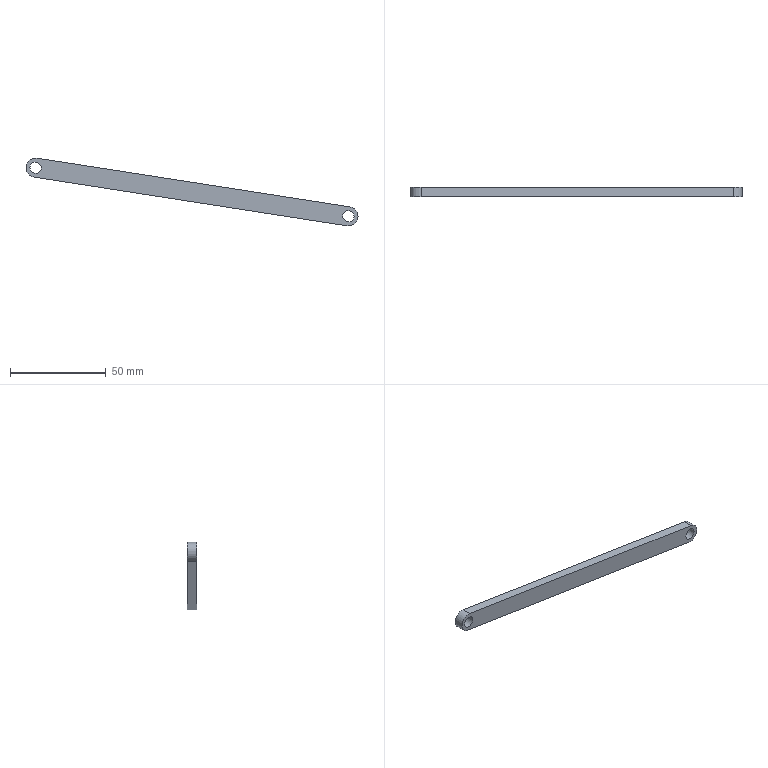Component | NX | 165 | 1 solid | 8 faces | box 173.04 x 5 x 35.33 mm | volume 8367 mm3 | plane 4 | cylinder 4 | commonest cylinder face diameters 10 x2 5.929 x2
STEP:
#1=CARTESIAN_POINT('',(0.,0.,0.));
#2=DIRECTION('',(0.,0.,1.));
#3=DIRECTION('',(1.,0.,0.));
#4=AXIS2_PLACEMENT_3D('',#1,#2,#3);
#5=CARTESIAN_POINT('',(-253.952,40.95,64.859));
#6=VERTEX_POINT('',#5);
#7=CARTESIAN_POINT('',(-90.907,40.95,39.531));
#8=VERTEX_POINT('',#7);
#9=CARTESIAN_POINT('',(-253.952,40.95,64.859));
#10=DIRECTION('',(0.9881,0.,-0.1535));
#11=VECTOR('',#10,1.);
#12=LINE('',#9,#11);
#13=CARTESIAN_POINT('',(-253.952,35.95,64.859));
#14=DIRECTION('',(0.1535,0.,0.9881));
#15=DIRECTION('',(0.9881,0.,-0.1535));
#16=AXIS2_PLACEMENT_3D('',#13,#14,#15);
#17=PLANE('',#16);
#18=CARTESIAN_POINT('',(0.,5.));
#19=DIRECTION('',(1.,0.));
#20=VECTOR('',#19,1.);
#21=LINE('',#18,#20);
#22=(GEOMETRIC_REPRESENTATION_CONTEXT(2)PARAMETRIC_REPRESENTATION_CONTEXT()REPRESENTATION_CONTEXT('',''));
#23=DEFINITIONAL_REPRESENTATION('',(#21),#22);
#24=PCURVE('',#17,#23);
#25=CARTESIAN_POINT('',(-91.675,40.95,34.591));
#26=DIRECTION('',(0.,1.,0.));
#27=DIRECTION('',(0.1535,0.,0.9881));
#28=AXIS2_PLACEMENT_3D('',#25,#26,#27);
#29=PLANE('',#28);
#30=CARTESIAN_POINT('',(5.,-165.));
#31=DIRECTION('',(0.,1.));
#32=VECTOR('',#31,1.);
#33=LINE('',#30,#32);
#34=(GEOMETRIC_REPRESENTATION_CONTEXT(2)PARAMETRIC_REPRESENTATION_CONTEXT()REPRESENTATION_CONTEXT('',''));
#35=DEFINITIONAL_REPRESENTATION('',(#33),#34);
#36=PCURVE('',#29,#35);
#37=SURFACE_CURVE('',#12,(#24,#36),.PCURVE_S1.);
#38=EDGE_CURVE('',#6,#8,#37,.T.);
#39=ORIENTED_EDGE('',*,*,#38,.F.);
#40=CARTESIAN_POINT('',(-253.952,35.95,64.859));
#41=VERTEX_POINT('',#40);
#42=CARTESIAN_POINT('',(-253.952,35.95,64.859));
#43=DIRECTION('',(0.,1.,0.));
#44=VECTOR('',#43,1.);
#45=LINE('',#42,#44);
#46=CARTESIAN_POINT('',(0.,0.));
#47=DIRECTION('',(0.,1.));
#48=VECTOR('',#47,1.);
#49=LINE('',#46,#48);
#50=(GEOMETRIC_REPRESENTATION_CONTEXT(2)PARAMETRIC_REPRESENTATION_CONTEXT()REPRESENTATION_CONTEXT('',''));
#51=DEFINITIONAL_REPRESENTATION('',(#49),#50);
#52=PCURVE('',#17,#51);
#53=CARTESIAN_POINT('',(-254.719,35.95,59.918));
#54=DIRECTION('',(0.,1.,0.));
#55=DIRECTION('',(0.1535,0.,0.9881));
#56=AXIS2_PLACEMENT_3D('',#53,#54,#55);
#57=CYLINDRICAL_SURFACE('',#56,5.);
#58=CARTESIAN_POINT('',(6.283,0.));
#59=DIRECTION('',(0.,1.));
#60=VECTOR('',#59,1.);
#61=LINE('',#58,#60);
#62=(GEOMETRIC_REPRESENTATION_CONTEXT(2)PARAMETRIC_REPRESENTATION_CONTEXT()REPRESENTATION_CONTEXT('',''));
#63=DEFINITIONAL_REPRESENTATION('',(#61),#62);
#64=PCURVE('',#57,#63);
#65=SURFACE_CURVE('',#45,(#52,#64),.PCURVE_S1.);
#66=EDGE_CURVE('',#41,#6,#65,.T.);
#67=ORIENTED_EDGE('',*,*,#66,.F.);
#68=CARTESIAN_POINT('',(-90.907,35.95,39.531));
#69=VERTEX_POINT('',#68);
#70=CARTESIAN_POINT('',(-253.952,35.95,64.859));
#71=DIRECTION('',(0.9881,0.,-0.1535));
#72=VECTOR('',#71,1.);
#73=LINE('',#70,#72);
#74=CARTESIAN_POINT('',(0.,0.));
#75=DIRECTION('',(1.,0.));
#76=VECTOR('',#75,1.);
#77=LINE('',#74,#76);
#78=(GEOMETRIC_REPRESENTATION_CONTEXT(2)PARAMETRIC_REPRESENTATION_CONTEXT()REPRESENTATION_CONTEXT('',''));
#79=DEFINITIONAL_REPRESENTATION('',(#77),#78);
#80=PCURVE('',#17,#79);
#81=CARTESIAN_POINT('',(-91.675,35.95,34.591));
#82=DIRECTION('',(0.,1.,0.));
#83=DIRECTION('',(0.1535,0.,0.9881));
#84=AXIS2_PLACEMENT_3D('',#81,#82,#83);
#85=PLANE('',#84);
#86=CARTESIAN_POINT('',(5.,-165.));
#87=DIRECTION('',(0.,1.));
#88=VECTOR('',#87,1.);
#89=LINE('',#86,#88);
#90=(GEOMETRIC_REPRESENTATION_CONTEXT(2)PARAMETRIC_REPRESENTATION_CONTEXT()REPRESENTATION_CONTEXT('',''));
#91=DEFINITIONAL_REPRESENTATION('',(#89),#90);
#92=PCURVE('',#85,#91);
#93=SURFACE_CURVE('',#73,(#80,#92),.PCURVE_S1.);
#94=EDGE_CURVE('',#41,#69,#93,.T.);
#95=ORIENTED_EDGE('',*,*,#94,.T.);
#96=CARTESIAN_POINT('',(-90.907,35.95,39.531));
#97=DIRECTION('',(0.,1.,0.));
#98=VECTOR('',#97,1.);
#99=LINE('',#96,#98);
#100=CARTESIAN_POINT('',(165.,0.));
#101=DIRECTION('',(0.,1.));
#102=VECTOR('',#101,1.);
#103=LINE('',#100,#102);
#104=(GEOMETRIC_REPRESENTATION_CONTEXT(2)PARAMETRIC_REPRESENTATION_CONTEXT()REPRESENTATION_CONTEXT('',''));
#105=DEFINITIONAL_REPRESENTATION('',(#103),#104);
#106=PCURVE('',#17,#105);
#107=CARTESIAN_POINT('',(-91.675,35.95,34.591));
#108=DIRECTION('',(0.,1.,0.));
#109=DIRECTION('',(0.1535,0.,0.9881));
#110=AXIS2_PLACEMENT_3D('',#107,#108,#109);
#111=CYLINDRICAL_SURFACE('',#110,5.);
#112=CARTESIAN_POINT('',(0.,0.));
#113=DIRECTION('',(0.,1.));
#114=VECTOR('',#113,1.);
#115=LINE('',#112,#114);
#116=(GEOMETRIC_REPRESENTATION_CONTEXT(2)PARAMETRIC_REPRESENTATION_CONTEXT()REPRESENTATION_CONTEXT('',''));
#117=DEFINITIONAL_REPRESENTATION('',(#115),#116);
#118=PCURVE('',#111,#117);
#119=SURFACE_CURVE('',#99,(#106,#118),.PCURVE_S1.);
#120=EDGE_CURVE('',#69,#8,#119,.T.);
#121=ORIENTED_EDGE('',*,*,#120,.T.);
#122=EDGE_LOOP('',(#39,#67,#95,#121));
#123=FACE_BOUND('',#122,.T.);
#124=ADVANCED_FACE('',(#123),#17,.T.);
#125=CARTESIAN_POINT('',(-92.442,40.95,29.65));
#126=VERTEX_POINT('',#125);
#127=CARTESIAN_POINT('',(-91.675,40.95,34.591));
#128=DIRECTION('',(0.,1.,0.));
#129=DIRECTION('',(0.1535,0.,0.9881));
#130=AXIS2_PLACEMENT_3D('',#127,#128,#129);
#131=CIRCLE('',#130,5.);
#132=CARTESIAN_POINT('',(0.,5.));
#133=DIRECTION('',(1.,0.));
#134=VECTOR('',#133,1.);
#135=LINE('',#132,#134);
#136=(GEOMETRIC_REPRESENTATION_CONTEXT(2)PARAMETRIC_REPRESENTATION_CONTEXT()REPRESENTATION_CONTEXT('',''));
#137=DEFINITIONAL_REPRESENTATION('',(#135),#136);
#138=PCURVE('',#111,#137);
#139=CARTESIAN_POINT('',(0.,0.));
#140=DIRECTION('',(1.,0.));
#141=AXIS2_PLACEMENT_2D('',#139,#140);
#142=CIRCLE('',#141,5.);
#143=(GEOMETRIC_REPRESENTATION_CONTEXT(2)PARAMETRIC_REPRESENTATION_CONTEXT()REPRESENTATION_CONTEXT('',''));
#144=DEFINITIONAL_REPRESENTATION('',(#142),#143);
#145=PCURVE('',#29,#144);
#146=SURFACE_CURVE('',#131,(#138,#145),.PCURVE_S1.);
#147=EDGE_CURVE('',#8,#126,#146,.T.);
#148=ORIENTED_EDGE('',*,*,#147,.F.);
#149=ORIENTED_EDGE('',*,*,#120,.F.);
#150=CARTESIAN_POINT('',(-92.442,35.95,29.65));
#151=VERTEX_POINT('',#150);
#152=CARTESIAN_POINT('',(-91.675,35.95,34.591));
#153=DIRECTION('',(0.,1.,0.));
#154=DIRECTION('',(0.1535,0.,0.9881));
#155=AXIS2_PLACEMENT_3D('',#152,#153,#154);
#156=CIRCLE('',#155,5.);
#157=CARTESIAN_POINT('',(0.,0.));
#158=DIRECTION('',(1.,0.));
#159=VECTOR('',#158,1.);
#160=LINE('',#157,#159);
#161=(GEOMETRIC_REPRESENTATION_CONTEXT(2)PARAMETRIC_REPRESENTATION_CONTEXT()REPRESENTATION_CONTEXT('',''));
#162=DEFINITIONAL_REPRESENTATION('',(#160),#161);
#163=PCURVE('',#111,#162);
#164=CARTESIAN_POINT('',(0.,0.));
#165=DIRECTION('',(1.,0.));
#166=AXIS2_PLACEMENT_2D('',#164,#165);
#167=CIRCLE('',#166,5.);
#168=(GEOMETRIC_REPRESENTATION_CONTEXT(2)PARAMETRIC_REPRESENTATION_CONTEXT()REPRESENTATION_CONTEXT('',''));
#169=DEFINITIONAL_REPRESENTATION('',(#167),#168);
#170=PCURVE('',#85,#169);
#171=SURFACE_CURVE('',#156,(#163,#170),.PCURVE_S1.);
#172=EDGE_CURVE('',#69,#151,#171,.T.);
#173=ORIENTED_EDGE('',*,*,#172,.T.);
#174=CARTESIAN_POINT('',(-92.442,35.95,29.65));
#175=DIRECTION('',(0.,1.,0.));
#176=VECTOR('',#175,1.);
#177=LINE('',#174,#176);
#178=CARTESIAN_POINT('',(3.142,0.));
#179=DIRECTION('',(0.,1.));
#180=VECTOR('',#179,1.);
#181=LINE('',#178,#180);
#182=(GEOMETRIC_REPRESENTATION_CONTEXT(2)PARAMETRIC_REPRESENTATION_CONTEXT()REPRESENTATION_CONTEXT('',''));
#183=DEFINITIONAL_REPRESENTATION('',(#181),#182);
#184=PCURVE('',#111,#183);
#185=CARTESIAN_POINT('',(-92.442,35.95,29.65));
#186=DIRECTION('',(-0.1535,0.,-0.9881));
#187=DIRECTION('',(-0.9881,0.,0.1535));
#188=AXIS2_PLACEMENT_3D('',#185,#186,#187);
#189=PLANE('',#188);
#190=CARTESIAN_POINT('',(0.,0.));
#191=DIRECTION('',(0.,1.));
#192=VECTOR('',#191,1.);
#193=LINE('',#190,#192);
#194=(GEOMETRIC_REPRESENTATION_CONTEXT(2)PARAMETRIC_REPRESENTATION_CONTEXT()REPRESENTATION_CONTEXT('',''));
#195=DEFINITIONAL_REPRESENTATION('',(#193),#194);
#196=PCURVE('',#189,#195);
#197=SURFACE_CURVE('',#177,(#184,#196),.PCURVE_S1.);
#198=EDGE_CURVE('',#151,#126,#197,.T.);
#199=ORIENTED_EDGE('',*,*,#198,.T.);
#200=EDGE_LOOP('',(#148,#149,#173,#199));
#201=FACE_BOUND('',#200,.T.);
#202=ADVANCED_FACE('',(#201),#111,.T.);
#203=CARTESIAN_POINT('',(-255.487,40.95,54.977));
#204=VERTEX_POINT('',#203);
#205=CARTESIAN_POINT('',(-92.442,40.95,29.65));
#206=DIRECTION('',(-0.9881,0.,0.1535));
#207=VECTOR('',#206,1.);
#208=LINE('',#205,#207);
#209=CARTESIAN_POINT('',(0.,5.));
#210=DIRECTION('',(1.,0.));
#211=VECTOR('',#210,1.);
#212=LINE('',#209,#211);
#213=(GEOMETRIC_REPRESENTATION_CONTEXT(2)PARAMETRIC_REPRESENTATION_CONTEXT()REPRESENTATION_CONTEXT('',''));
#214=DEFINITIONAL_REPRESENTATION('',(#212),#213);
#215=PCURVE('',#189,#214);
#216=CARTESIAN_POINT('',(-5.,0.));
#217=DIRECTION('',(0.,-1.));
#218=VECTOR('',#217,1.);
#219=LINE('',#216,#218);
#220=(GEOMETRIC_REPRESENTATION_CONTEXT(2)PARAMETRIC_REPRESENTATION_CONTEXT()REPRESENTATION_CONTEXT('',''));
#221=DEFINITIONAL_REPRESENTATION('',(#219),#220);
#222=PCURVE('',#29,#221);
#223=SURFACE_CURVE('',#208,(#215,#222),.PCURVE_S1.);
#224=EDGE_CURVE('',#126,#204,#223,.T.);
#225=ORIENTED_EDGE('',*,*,#224,.F.);
#226=ORIENTED_EDGE('',*,*,#198,.F.);
#227=CARTESIAN_POINT('',(-255.487,35.95,54.977));
#228=VERTEX_POINT('',#227);
#229=CARTESIAN_POINT('',(-92.442,35.95,29.65));
#230=DIRECTION('',(-0.9881,0.,0.1535));
#231=VECTOR('',#230,1.);
#232=LINE('',#229,#231);
#233=CARTESIAN_POINT('',(0.,0.));
#234=DIRECTION('',(1.,0.));
#235=VECTOR('',#234,1.);
#236=LINE('',#233,#235);
#237=(GEOMETRIC_REPRESENTATION_CONTEXT(2)PARAMETRIC_REPRESENTATION_CONTEXT()REPRESENTATION_CONTEXT('',''));
#238=DEFINITIONAL_REPRESENTATION('',(#236),#237);
#239=PCURVE('',#189,#238);
#240=CARTESIAN_POINT('',(-5.,0.));
#241=DIRECTION('',(0.,-1.));
#242=VECTOR('',#241,1.);
#243=LINE('',#240,#242);
#244=(GEOMETRIC_REPRESENTATION_CONTEXT(2)PARAMETRIC_REPRESENTATION_CONTEXT()REPRESENTATION_CONTEXT('',''));
#245=DEFINITIONAL_REPRESENTATION('',(#243),#244);
#246=PCURVE('',#85,#245);
#247=SURFACE_CURVE('',#232,(#239,#246),.PCURVE_S1.);
#248=EDGE_CURVE('',#151,#228,#247,.T.);
#249=ORIENTED_EDGE('',*,*,#248,.T.);
#250=CARTESIAN_POINT('',(-255.487,35.95,54.977));
#251=DIRECTION('',(0.,1.,0.));
#252=VECTOR('',#251,1.);
#253=LINE('',#250,#252);
#254=CARTESIAN_POINT('',(165.,0.));
#255=DIRECTION('',(0.,1.));
#256=VECTOR('',#255,1.);
#257=LINE('',#254,#256);
#258=(GEOMETRIC_REPRESENTATION_CONTEXT(2)PARAMETRIC_REPRESENTATION_CONTEXT()REPRESENTATION_CONTEXT('',''));
#259=DEFINITIONAL_REPRESENTATION('',(#257),#258);
#260=PCURVE('',#189,#259);
#261=CARTESIAN_POINT('',(3.142,0.));
#262=DIRECTION('',(0.,1.));
#263=VECTOR('',#262,1.);
#264=LINE('',#261,#263);
#265=(GEOMETRIC_REPRESENTATION_CONTEXT(2)PARAMETRIC_REPRESENTATION_CONTEXT()REPRESENTATION_CONTEXT('',''));
#266=DEFINITIONAL_REPRESENTATION('',(#264),#265);
#267=PCURVE('',#57,#266);
#268=SURFACE_CURVE('',#253,(#260,#267),.PCURVE_S1.);
#269=EDGE_CURVE('',#228,#204,#268,.T.);
#270=ORIENTED_EDGE('',*,*,#269,.T.);
#271=EDGE_LOOP('',(#225,#226,#249,#270));
#272=FACE_BOUND('',#271,.T.);
#273=ADVANCED_FACE('',(#272),#189,.T.);
#274=CARTESIAN_POINT('',(-254.264,35.95,62.847));
#275=VERTEX_POINT('',#274);
#276=CARTESIAN_POINT('',(-254.719,35.95,59.918));
#277=DIRECTION('',(0.,1.,0.));
#278=DIRECTION('',(0.1535,0.,0.9881));
#279=AXIS2_PLACEMENT_3D('',#276,#277,#278);
#280=CIRCLE('',#279,2.964);
#281=CARTESIAN_POINT('',(-254.719,35.95,59.918));
#282=DIRECTION('',(0.,1.,0.));
#283=DIRECTION('',(0.1535,0.,0.9881));
#284=AXIS2_PLACEMENT_3D('',#281,#282,#283);
#285=CYLINDRICAL_SURFACE('',#284,2.964);
#286=CARTESIAN_POINT('',(0.,0.));
#287=DIRECTION('',(1.,0.));
#288=VECTOR('',#287,1.);
#289=LINE('',#286,#288);
#290=(GEOMETRIC_REPRESENTATION_CONTEXT(2)PARAMETRIC_REPRESENTATION_CONTEXT()REPRESENTATION_CONTEXT('',''));
#291=DEFINITIONAL_REPRESENTATION('',(#289),#290);
#292=PCURVE('',#285,#291);
#293=CARTESIAN_POINT('',(0.,-165.));
#294=DIRECTION('',(1.,-0.));
#295=AXIS2_PLACEMENT_2D('',#293,#294);
#296=CIRCLE('',#295,2.964);
#297=(GEOMETRIC_REPRESENTATION_CONTEXT(2)PARAMETRIC_REPRESENTATION_CONTEXT()REPRESENTATION_CONTEXT('',''));
#298=DEFINITIONAL_REPRESENTATION('',(#296),#297);
#299=PCURVE('',#85,#298);
#300=SURFACE_CURVE('',#280,(#292,#299),.PCURVE_S1.);
#301=EDGE_CURVE('',#275,#275,#300,.T.);
#302=ORIENTED_EDGE('',*,*,#301,.T.);
#303=CARTESIAN_POINT('',(-254.264,40.95,62.847));
#304=VERTEX_POINT('',#303);
#305=CARTESIAN_POINT('',(-254.264,35.95,62.847));
#306=CARTESIAN_POINT('',(-254.264,40.95,62.847));
#307=B_SPLINE_CURVE_WITH_KNOTS('',1,(#305,#306),.UNSPECIFIED.,.F.,.F.,(2,2),(0.,5.),.PIECEWISE_BEZIER_KNOTS.);
#308=CARTESIAN_POINT('',(6.283,0.));
#309=DIRECTION('',(0.,1.));
#310=VECTOR('',#309,1.);
#311=LINE('',#308,#310);
#312=(GEOMETRIC_REPRESENTATION_CONTEXT(2)PARAMETRIC_REPRESENTATION_CONTEXT()REPRESENTATION_CONTEXT('',''));
#313=DEFINITIONAL_REPRESENTATION('',(#311),#312);
#314=PCURVE('',#285,#313);
#315=CARTESIAN_POINT('',(0.,0.));
#316=DIRECTION('',(0.,1.));
#317=VECTOR('',#316,1.);
#318=LINE('',#315,#317);
#319=(GEOMETRIC_REPRESENTATION_CONTEXT(2)PARAMETRIC_REPRESENTATION_CONTEXT()REPRESENTATION_CONTEXT('',''));
#320=DEFINITIONAL_REPRESENTATION('',(#318),#319);
#321=PCURVE('',#285,#320);
#322=SEAM_CURVE('',#307,(#314,#321),.PCURVE_S1.);
#323=EDGE_CURVE('',#275,#304,#322,.T.);
#324=ORIENTED_EDGE('',*,*,#323,.T.);
#325=CARTESIAN_POINT('',(-254.719,40.95,59.918));
#326=DIRECTION('',(0.,1.,0.));
#327=DIRECTION('',(0.1535,0.,0.9881));
#328=AXIS2_PLACEMENT_3D('',#325,#326,#327);
#329=CIRCLE('',#328,2.964);
#330=CARTESIAN_POINT('',(0.,5.));
#331=DIRECTION('',(1.,0.));
#332=VECTOR('',#331,1.);
#333=LINE('',#330,#332);
#334=(GEOMETRIC_REPRESENTATION_CONTEXT(2)PARAMETRIC_REPRESENTATION_CONTEXT()REPRESENTATION_CONTEXT('',''));
#335=DEFINITIONAL_REPRESENTATION('',(#333),#334);
#336=PCURVE('',#285,#335);
#337=CARTESIAN_POINT('',(0.,-165.));
#338=DIRECTION('',(1.,-0.));
#339=AXIS2_PLACEMENT_2D('',#337,#338);
#340=CIRCLE('',#339,2.964);
#341=(GEOMETRIC_REPRESENTATION_CONTEXT(2)PARAMETRIC_REPRESENTATION_CONTEXT()REPRESENTATION_CONTEXT('',''));
#342=DEFINITIONAL_REPRESENTATION('',(#340),#341);
#343=PCURVE('',#29,#342);
#344=SURFACE_CURVE('',#329,(#336,#343),.PCURVE_S1.);
#345=EDGE_CURVE('',#304,#304,#344,.T.);
#346=ORIENTED_EDGE('',*,*,#345,.F.);
#347=ORIENTED_EDGE('',*,*,#323,.F.);
#348=EDGE_LOOP('',(#302,#324,#346,#347));
#349=FACE_BOUND('',#348,.F.);
#350=ADVANCED_FACE('',(#349),#285,.F.);
#351=CARTESIAN_POINT('',(-254.719,40.95,59.918));
#352=DIRECTION('',(0.,1.,0.));
#353=DIRECTION('',(0.1535,0.,0.9881));
#354=AXIS2_PLACEMENT_3D('',#351,#352,#353);
#355=CIRCLE('',#354,5.);
#356=CARTESIAN_POINT('',(0.,5.));
#357=DIRECTION('',(1.,0.));
#358=VECTOR('',#357,1.);
#359=LINE('',#356,#358);
#360=(GEOMETRIC_REPRESENTATION_CONTEXT(2)PARAMETRIC_REPRESENTATION_CONTEXT()REPRESENTATION_CONTEXT('',''));
#361=DEFINITIONAL_REPRESENTATION('',(#359),#360);
#362=PCURVE('',#57,#361);
#363=CARTESIAN_POINT('',(0.,-165.));
#364=DIRECTION('',(1.,0.));
#365=AXIS2_PLACEMENT_2D('',#363,#364);
#366=CIRCLE('',#365,5.);
#367=(GEOMETRIC_REPRESENTATION_CONTEXT(2)PARAMETRIC_REPRESENTATION_CONTEXT()REPRESENTATION_CONTEXT('',''));
#368=DEFINITIONAL_REPRESENTATION('',(#366),#367);
#369=PCURVE('',#29,#368);
#370=SURFACE_CURVE('',#355,(#362,#369),.PCURVE_S1.);
#371=EDGE_CURVE('',#204,#6,#370,.T.);
#372=ORIENTED_EDGE('',*,*,#371,.F.);
#373=ORIENTED_EDGE('',*,*,#269,.F.);
#374=CARTESIAN_POINT('',(-254.719,35.95,59.918));
#375=DIRECTION('',(0.,1.,0.));
#376=DIRECTION('',(0.1535,0.,0.9881));
#377=AXIS2_PLACEMENT_3D('',#374,#375,#376);
#378=CIRCLE('',#377,5.);
#379=CARTESIAN_POINT('',(0.,0.));
#380=DIRECTION('',(1.,0.));
#381=VECTOR('',#380,1.);
#382=LINE('',#379,#381);
#383=(GEOMETRIC_REPRESENTATION_CONTEXT(2)PARAMETRIC_REPRESENTATION_CONTEXT()REPRESENTATION_CONTEXT('',''));
#384=DEFINITIONAL_REPRESENTATION('',(#382),#383);
#385=PCURVE('',#57,#384);
#386=CARTESIAN_POINT('',(0.,-165.));
#387=DIRECTION('',(1.,0.));
#388=AXIS2_PLACEMENT_2D('',#386,#387);
#389=CIRCLE('',#388,5.);
#390=(GEOMETRIC_REPRESENTATION_CONTEXT(2)PARAMETRIC_REPRESENTATION_CONTEXT()REPRESENTATION_CONTEXT('',''));
#391=DEFINITIONAL_REPRESENTATION('',(#389),#390);
#392=PCURVE('',#85,#391);
#393=SURFACE_CURVE('',#378,(#385,#392),.PCURVE_S1.);
#394=EDGE_CURVE('',#228,#41,#393,.T.);
#395=ORIENTED_EDGE('',*,*,#394,.T.);
#396=ORIENTED_EDGE('',*,*,#66,.T.);
#397=EDGE_LOOP('',(#372,#373,#395,#396));
#398=FACE_BOUND('',#397,.T.);
#399=ADVANCED_FACE('',(#398),#57,.T.);
#400=CARTESIAN_POINT('',(-91.22,35.95,37.52));
#401=VERTEX_POINT('',#400);
#402=CARTESIAN_POINT('',(-91.675,35.95,34.591));
#403=DIRECTION('',(0.,1.,0.));
#404=DIRECTION('',(0.1535,0.,0.9881));
#405=AXIS2_PLACEMENT_3D('',#402,#403,#404);
#406=CIRCLE('',#405,2.964);
#407=CARTESIAN_POINT('',(-91.675,35.95,34.591));
#408=DIRECTION('',(0.,1.,0.));
#409=DIRECTION('',(0.1535,0.,0.9881));
#410=AXIS2_PLACEMENT_3D('',#407,#408,#409);
#411=CYLINDRICAL_SURFACE('',#410,2.964);
#412=CARTESIAN_POINT('',(0.,0.));
#413=DIRECTION('',(1.,0.));
#414=VECTOR('',#413,1.);
#415=LINE('',#412,#414);
#416=(GEOMETRIC_REPRESENTATION_CONTEXT(2)PARAMETRIC_REPRESENTATION_CONTEXT()REPRESENTATION_CONTEXT('',''));
#417=DEFINITIONAL_REPRESENTATION('',(#415),#416);
#418=PCURVE('',#411,#417);
#419=CARTESIAN_POINT('',(0.,0.));
#420=DIRECTION('',(1.,-0.));
#421=AXIS2_PLACEMENT_2D('',#419,#420);
#422=CIRCLE('',#421,2.964);
#423=(GEOMETRIC_REPRESENTATION_CONTEXT(2)PARAMETRIC_REPRESENTATION_CONTEXT()REPRESENTATION_CONTEXT('',''));
#424=DEFINITIONAL_REPRESENTATION('',(#422),#423);
#425=PCURVE('',#85,#424);
#426=SURFACE_CURVE('',#406,(#418,#425),.PCURVE_S1.);
#427=EDGE_CURVE('',#401,#401,#426,.T.);
#428=ORIENTED_EDGE('',*,*,#427,.T.);
#429=CARTESIAN_POINT('',(-91.22,40.95,37.52));
#430=VERTEX_POINT('',#429);
#431=CARTESIAN_POINT('',(-91.22,35.95,37.52));
#432=CARTESIAN_POINT('',(-91.22,40.95,37.52));
#433=B_SPLINE_CURVE_WITH_KNOTS('',1,(#431,#432),.UNSPECIFIED.,.F.,.F.,(2,2),(0.,5.),.PIECEWISE_BEZIER_KNOTS.);
#434=CARTESIAN_POINT('',(6.283,0.));
#435=DIRECTION('',(0.,1.));
#436=VECTOR('',#435,1.);
#437=LINE('',#434,#436);
#438=(GEOMETRIC_REPRESENTATION_CONTEXT(2)PARAMETRIC_REPRESENTATION_CONTEXT()REPRESENTATION_CONTEXT('',''));
#439=DEFINITIONAL_REPRESENTATION('',(#437),#438);
#440=PCURVE('',#411,#439);
#441=CARTESIAN_POINT('',(0.,0.));
#442=DIRECTION('',(0.,1.));
#443=VECTOR('',#442,1.);
#444=LINE('',#441,#443);
#445=(GEOMETRIC_REPRESENTATION_CONTEXT(2)PARAMETRIC_REPRESENTATION_CONTEXT()REPRESENTATION_CONTEXT('',''));
#446=DEFINITIONAL_REPRESENTATION('',(#444),#445);
#447=PCURVE('',#411,#446);
#448=SEAM_CURVE('',#433,(#440,#447),.PCURVE_S1.);
#449=EDGE_CURVE('',#401,#430,#448,.T.);
#450=ORIENTED_EDGE('',*,*,#449,.T.);
#451=CARTESIAN_POINT('',(-91.675,40.95,34.591));
#452=DIRECTION('',(0.,1.,0.));
#453=DIRECTION('',(0.1535,0.,0.9881));
#454=AXIS2_PLACEMENT_3D('',#451,#452,#453);
#455=CIRCLE('',#454,2.964);
#456=CARTESIAN_POINT('',(0.,5.));
#457=DIRECTION('',(1.,0.));
#458=VECTOR('',#457,1.);
#459=LINE('',#456,#458);
#460=(GEOMETRIC_REPRESENTATION_CONTEXT(2)PARAMETRIC_REPRESENTATION_CONTEXT()REPRESENTATION_CONTEXT('',''));
#461=DEFINITIONAL_REPRESENTATION('',(#459),#460);
#462=PCURVE('',#411,#461);
#463=CARTESIAN_POINT('',(0.,0.));
#464=DIRECTION('',(1.,-0.));
#465=AXIS2_PLACEMENT_2D('',#463,#464);
#466=CIRCLE('',#465,2.964);
#467=(GEOMETRIC_REPRESENTATION_CONTEXT(2)PARAMETRIC_REPRESENTATION_CONTEXT()REPRESENTATION_CONTEXT('',''));
#468=DEFINITIONAL_REPRESENTATION('',(#466),#467);
#469=PCURVE('',#29,#468);
#470=SURFACE_CURVE('',#455,(#462,#469),.PCURVE_S1.);
#471=EDGE_CURVE('',#430,#430,#470,.T.);
#472=ORIENTED_EDGE('',*,*,#471,.F.);
#473=ORIENTED_EDGE('',*,*,#449,.F.);
#474=EDGE_LOOP('',(#428,#450,#472,#473));
#475=FACE_BOUND('',#474,.F.);
#476=ADVANCED_FACE('',(#475),#411,.F.);
#477=ORIENTED_EDGE('',*,*,#94,.F.);
#478=ORIENTED_EDGE('',*,*,#394,.F.);
#479=ORIENTED_EDGE('',*,*,#248,.F.);
#480=ORIENTED_EDGE('',*,*,#172,.F.);
#481=EDGE_LOOP('',(#477,#478,#479,#480));
#482=FACE_BOUND('',#481,.T.);
#483=ORIENTED_EDGE('',*,*,#301,.T.);
#484=EDGE_LOOP('',(#483));
#485=FACE_BOUND('',#484,.T.);
#486=ORIENTED_EDGE('',*,*,#427,.T.);
#487=EDGE_LOOP('',(#486));
#488=FACE_BOUND('',#487,.T.);
#489=ADVANCED_FACE('',(#482,#485,#488),#85,.F.);
#490=ORIENTED_EDGE('',*,*,#38,.T.);
#491=ORIENTED_EDGE('',*,*,#147,.T.);
#492=ORIENTED_EDGE('',*,*,#224,.T.);
#493=ORIENTED_EDGE('',*,*,#371,.T.);
#494=EDGE_LOOP('',(#490,#491,#492,#493));
#495=FACE_BOUND('',#494,.T.);
#496=ORIENTED_EDGE('',*,*,#345,.F.);
#497=EDGE_LOOP('',(#496));
#498=FACE_BOUND('',#497,.T.);
#499=ORIENTED_EDGE('',*,*,#471,.F.);
#500=EDGE_LOOP('',(#499));
#501=FACE_BOUND('',#500,.T.);
#502=ADVANCED_FACE('',(#495,#498,#501),#29,.T.);
#503=CLOSED_SHELL('',(#124,#202,#273,#350,#399,#476,#489,#502));
#504=MANIFOLD_SOLID_BREP('',#503);
#505=(LENGTH_UNIT()NAMED_UNIT(*)SI_UNIT(.MILLI.,.METRE.));
#506=UNCERTAINTY_MEASURE_WITH_UNIT(LENGTH_MEASURE(0.000002),#505,'','');
#507=(NAMED_UNIT(*)PLANE_ANGLE_UNIT()SI_UNIT($,.RADIAN.));
#508=(NAMED_UNIT(*)SI_UNIT($,.STERADIAN.)SOLID_ANGLE_UNIT());
#509=(GEOMETRIC_REPRESENTATION_CONTEXT(3)GLOBAL_UNCERTAINTY_ASSIGNED_CONTEXT((#506))GLOBAL_UNIT_ASSIGNED_CONTEXT((#505,#507,#508))REPRESENTATION_CONTEXT('',''));
#510=ADVANCED_BREP_SHAPE_REPRESENTATION('',(#4,#504),#509);